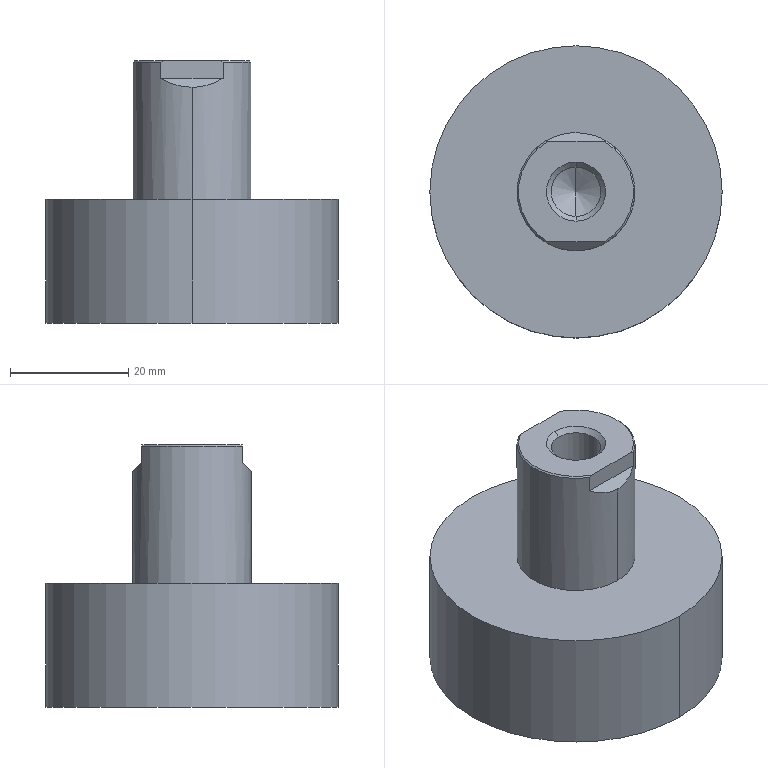Component | NX | SDAS-50X55_R | 1 solid | 19 faces | volume 46672 mm3 | plane 7 | cone 6 | cylinder 6 | commonest cylinder face diameters 8.376 x2 20 x2 49.5 x2